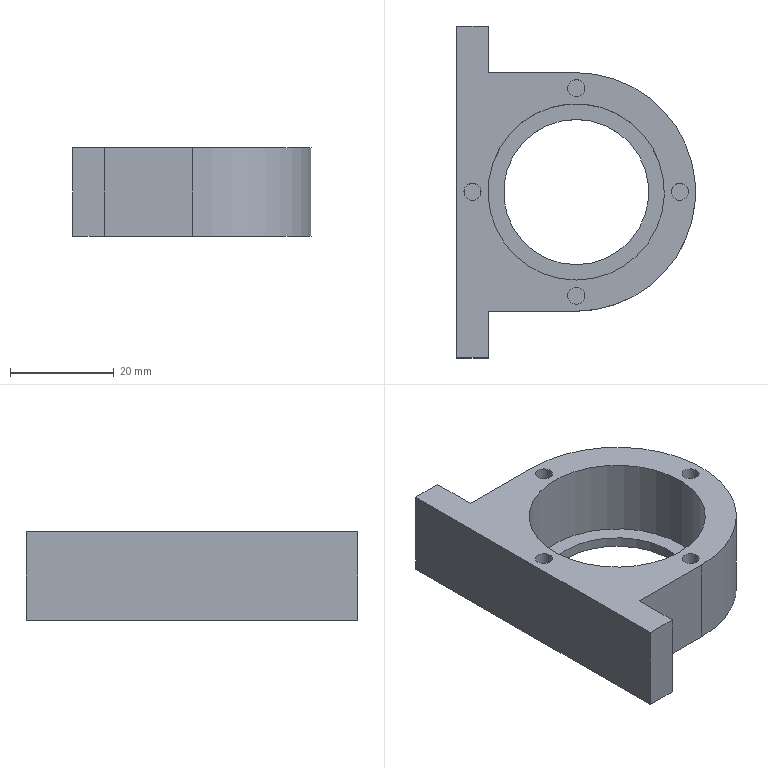Component | NX | BEARING_BLOCK | 1 solid | 21 faces | volume 18687 mm3 | plane 14 | cylinder 7 | commonest cylinder face diameters 3.3 x4 28 x1 46 x1 34 x1